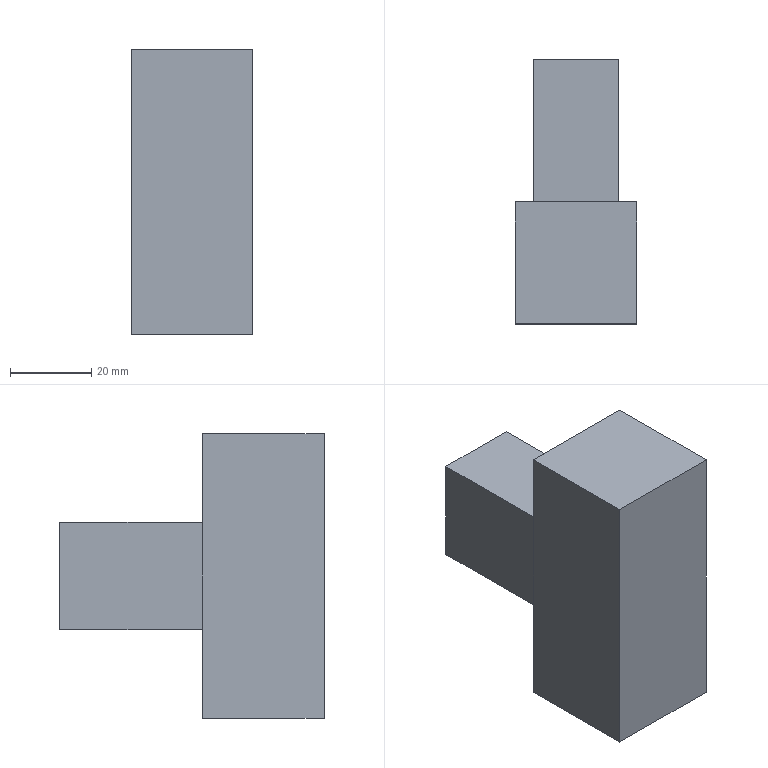Component | SolidWorks | HH54PIntermediateRelay-4 | 1 solid | 11 faces | box 30 x 65 x 70 mm | volume 82477 mm3 | plane 11
build123d program:
from build123d import *

# Parameters (mm, degrees)
SKETCH1_W           = 30
SKETCH1_H           = 70
BOSS_EXTRUDE1_DEPTH = 30
SKETCH2_W           = 21
SKETCH2_H           = 26.5
BOSS_EXTRUDE2_DEPTH = 35


with BuildPart() as part:
    # Sketch1 → Boss-Extrude1 (new body)
    with BuildSketch(Plane.XY):
        with Locations((-5.463, -8.36)):
            Rectangle(SKETCH1_W, SKETCH1_H)
    extrude(amount=BOSS_EXTRUDE1_DEPTH)

    # Sketch2 → Boss-Extrude2 (add)
    with BuildSketch(Plane.XY.offset(30)):
        with Locations((-5.463, -8.36)):
            Rectangle(SKETCH2_W, SKETCH2_H)
    extrude(amount=BOSS_EXTRUDE2_DEPTH)


solid = part.part

# Placed as in the assembly
solid = solid.moved(Location((276.983, -49.298, 757.449), (-90, 0, 0)))
STEP:
#1=COLOUR_RGB('',0.7922,0.8196,0.9333);
#2=FILL_AREA_STYLE_COLOUR('',#1);
#3=FILL_AREA_STYLE('',(#2));
#4=SURFACE_STYLE_FILL_AREA(#3);
#5=SURFACE_SIDE_STYLE('',(#4));
#6=SURFACE_STYLE_USAGE(.BOTH.,#5);
#7=PRESENTATION_STYLE_ASSIGNMENT((#6));
#8=CARTESIAN_POINT('',(10.099,-0.7598,28.772));
#9=VERTEX_POINT('',#8);
#10=CARTESIAN_POINT('',(10.099,-0.7598,31.528));
#11=VERTEX_POINT('',#10);
#12=CARTESIAN_POINT('',(10.099,-0.7598,28.772));
#13=DIRECTION('',(0.,0.,1.));
#14=VECTOR('',#13,39.37);
#15=LINE('',#12,#14);
#16=EDGE_CURVE('',#9,#11,#15,.T.);
#17=ORIENTED_EDGE('',*,*,#16,.T.);
#18=CARTESIAN_POINT('',(11.28,-0.7598,31.528));
#19=VERTEX_POINT('',#18);
#20=CARTESIAN_POINT('',(10.099,-0.7598,31.528));
#21=DIRECTION('',(1.,0.,0.));
#22=VECTOR('',#21,39.37);
#23=LINE('',#20,#22);
#24=EDGE_CURVE('',#11,#19,#23,.T.);
#25=ORIENTED_EDGE('',*,*,#24,.T.);
#26=CARTESIAN_POINT('',(11.28,-0.7598,28.772));
#27=VERTEX_POINT('',#26);
#28=CARTESIAN_POINT('',(11.28,-0.7598,28.772));
#29=DIRECTION('',(-0.,-0.,-1.));
#30=VECTOR('',#29,39.37);
#31=LINE('',#28,#30);
#32=EDGE_CURVE('',#19,#27,#31,.T.);
#33=ORIENTED_EDGE('',*,*,#32,.T.);
#34=CARTESIAN_POINT('',(10.099,-0.7598,28.772));
#35=DIRECTION('',(-1.,0.,0.));
#36=VECTOR('',#35,39.37);
#37=LINE('',#34,#36);
#38=EDGE_CURVE('',#27,#9,#37,.T.);
#39=ORIENTED_EDGE('',*,*,#38,.T.);
#40=EDGE_LOOP('',(#17,#25,#33,#39));
#41=FACE_OUTER_BOUND('',#40,.T.);
#42=CARTESIAN_POINT('',(10.276,-0.7598,30.672));
#43=VERTEX_POINT('',#42);
#44=CARTESIAN_POINT('',(11.103,-0.7598,30.672));
#45=VERTEX_POINT('',#44);
#46=CARTESIAN_POINT('',(10.276,-0.7598,30.672));
#47=DIRECTION('',(1.,0.,0.));
#48=VECTOR('',#47,39.37);
#49=LINE('',#46,#48);
#50=EDGE_CURVE('',#43,#45,#49,.T.);
#51=ORIENTED_EDGE('',*,*,#50,.F.);
#52=CARTESIAN_POINT('',(10.276,-0.7598,29.628));
#53=VERTEX_POINT('',#52);
#54=CARTESIAN_POINT('',(10.276,-0.7598,29.628));
#55=DIRECTION('',(0.,0.,1.));
#56=VECTOR('',#55,39.37);
#57=LINE('',#54,#56);
#58=EDGE_CURVE('',#53,#43,#57,.T.);
#59=ORIENTED_EDGE('',*,*,#58,.F.);
#60=CARTESIAN_POINT('',(11.103,-0.7598,29.628));
#61=VERTEX_POINT('',#60);
#62=CARTESIAN_POINT('',(10.276,-0.7598,29.628));
#63=DIRECTION('',(-1.,0.,0.));
#64=VECTOR('',#63,39.37);
#65=LINE('',#62,#64);
#66=EDGE_CURVE('',#61,#53,#65,.T.);
#67=ORIENTED_EDGE('',*,*,#66,.F.);
#68=CARTESIAN_POINT('',(11.103,-0.7598,29.628));
#69=DIRECTION('',(-0.,-0.,-1.));
#70=VECTOR('',#69,39.37);
#71=LINE('',#68,#70);
#72=EDGE_CURVE('',#45,#61,#71,.T.);
#73=ORIENTED_EDGE('',*,*,#72,.F.);
#74=EDGE_LOOP('',(#51,#59,#67,#73));
#75=FACE_BOUND('',#74,.T.);
#76=CARTESIAN_POINT('',(10.905,-0.7598,29.821));
#77=DIRECTION('',(0.,1.,-0.));
#78=DIRECTION('',(1.,0.,0.));
#79=AXIS2_PLACEMENT_3D('',#76,#77,#78);
#80=PLANE('',#79);
#81=ADVANCED_FACE('',(#41,#75),#80,.T.);
#82=CARTESIAN_POINT('',(10.099,-1.941,28.772));
#83=VERTEX_POINT('',#82);
#84=CARTESIAN_POINT('',(10.099,-1.941,31.528));
#85=VERTEX_POINT('',#84);
#86=CARTESIAN_POINT('',(10.099,-1.941,28.772));
#87=DIRECTION('',(0.,0.,1.));
#88=VECTOR('',#87,39.37);
#89=LINE('',#86,#88);
#90=EDGE_CURVE('',#83,#85,#89,.T.);
#91=ORIENTED_EDGE('',*,*,#90,.T.);
#92=CARTESIAN_POINT('',(10.099,-0.7598,31.528));
#93=DIRECTION('',(0.,-1.,0.));
#94=VECTOR('',#93,39.37);
#95=LINE('',#92,#94);
#96=EDGE_CURVE('',#11,#85,#95,.T.);
#97=ORIENTED_EDGE('',*,*,#96,.F.);
#98=ORIENTED_EDGE('',*,*,#16,.F.);
#99=CARTESIAN_POINT('',(10.099,-0.7598,28.772));
#100=DIRECTION('',(0.,-1.,0.));
#101=VECTOR('',#100,39.37);
#102=LINE('',#99,#101);
#103=EDGE_CURVE('',#9,#83,#102,.T.);
#104=ORIENTED_EDGE('',*,*,#103,.T.);
#105=EDGE_LOOP('',(#91,#97,#98,#104));
#106=FACE_OUTER_BOUND('',#105,.T.);
#107=CARTESIAN_POINT('',(10.099,-0.7598,28.772));
#108=DIRECTION('',(1.,0.,0.));
#109=DIRECTION('',(0.,-1.,0.));
#110=AXIS2_PLACEMENT_3D('',#107,#108,#109);
#111=PLANE('',#110);
#112=ADVANCED_FACE('',(#106),#111,.F.);
#113=CARTESIAN_POINT('',(11.28,-1.941,31.528));
#114=VERTEX_POINT('',#113);
#115=CARTESIAN_POINT('',(10.099,-1.941,31.528));
#116=DIRECTION('',(1.,0.,0.));
#117=VECTOR('',#116,39.37);
#118=LINE('',#115,#117);
#119=EDGE_CURVE('',#85,#114,#118,.T.);
#120=ORIENTED_EDGE('',*,*,#119,.T.);
#121=CARTESIAN_POINT('',(11.28,-0.7598,31.528));
#122=DIRECTION('',(0.,-1.,0.));
#123=VECTOR('',#122,39.37);
#124=LINE('',#121,#123);
#125=EDGE_CURVE('',#19,#114,#124,.T.);
#126=ORIENTED_EDGE('',*,*,#125,.F.);
#127=ORIENTED_EDGE('',*,*,#24,.F.);
#128=ORIENTED_EDGE('',*,*,#96,.T.);
#129=EDGE_LOOP('',(#120,#126,#127,#128));
#130=FACE_OUTER_BOUND('',#129,.T.);
#131=CARTESIAN_POINT('',(10.099,-0.7598,31.528));
#132=DIRECTION('',(0.,-0.,-1.));
#133=DIRECTION('',(0.,1.,-0.));
#134=AXIS2_PLACEMENT_3D('',#131,#132,#133);
#135=PLANE('',#134);
#136=ADVANCED_FACE('',(#130),#135,.F.);
#137=CARTESIAN_POINT('',(11.28,-1.941,28.772));
#138=VERTEX_POINT('',#137);
#139=CARTESIAN_POINT('',(11.28,-1.941,28.772));
#140=DIRECTION('',(-0.,-0.,-1.));
#141=VECTOR('',#140,39.37);
#142=LINE('',#139,#141);
#143=EDGE_CURVE('',#114,#138,#142,.T.);
#144=ORIENTED_EDGE('',*,*,#143,.T.);
#145=CARTESIAN_POINT('',(11.28,-0.7598,28.772));
#146=DIRECTION('',(0.,-1.,0.));
#147=VECTOR('',#146,39.37);
#148=LINE('',#145,#147);
#149=EDGE_CURVE('',#27,#138,#148,.T.);
#150=ORIENTED_EDGE('',*,*,#149,.F.);
#151=ORIENTED_EDGE('',*,*,#32,.F.);
#152=ORIENTED_EDGE('',*,*,#125,.T.);
#153=EDGE_LOOP('',(#144,#150,#151,#152));
#154=FACE_OUTER_BOUND('',#153,.T.);
#155=CARTESIAN_POINT('',(11.28,-0.7598,28.772));
#156=DIRECTION('',(-1.,0.,0.));
#157=DIRECTION('',(0.,0.,1.));
#158=AXIS2_PLACEMENT_3D('',#155,#156,#157);
#159=PLANE('',#158);
#160=ADVANCED_FACE('',(#154),#159,.F.);
#161=CARTESIAN_POINT('',(10.099,-1.941,28.772));
#162=DIRECTION('',(-1.,0.,0.));
#163=VECTOR('',#162,39.37);
#164=LINE('',#161,#163);
#165=EDGE_CURVE('',#138,#83,#164,.T.);
#166=ORIENTED_EDGE('',*,*,#165,.T.);
#167=ORIENTED_EDGE('',*,*,#103,.F.);
#168=ORIENTED_EDGE('',*,*,#38,.F.);
#169=ORIENTED_EDGE('',*,*,#149,.T.);
#170=EDGE_LOOP('',(#166,#167,#168,#169));
#171=FACE_OUTER_BOUND('',#170,.T.);
#172=CARTESIAN_POINT('',(10.099,-0.7598,28.772));
#173=DIRECTION('',(0.,0.,1.));
#174=DIRECTION('',(0.,-1.,0.));
#175=AXIS2_PLACEMENT_3D('',#172,#173,#174);
#176=PLANE('',#175);
#177=ADVANCED_FACE('',(#171),#176,.F.);
#178=ORIENTED_EDGE('',*,*,#90,.F.);
#179=ORIENTED_EDGE('',*,*,#165,.F.);
#180=ORIENTED_EDGE('',*,*,#143,.F.);
#181=ORIENTED_EDGE('',*,*,#119,.F.);
#182=EDGE_LOOP('',(#178,#179,#180,#181));
#183=FACE_OUTER_BOUND('',#182,.T.);
#184=CARTESIAN_POINT('',(10.905,-1.941,29.821));
#185=DIRECTION('',(0.,1.,-0.));
#186=DIRECTION('',(1.,0.,0.));
#187=AXIS2_PLACEMENT_3D('',#184,#185,#186);
#188=PLANE('',#187);
#189=ADVANCED_FACE('',(#183),#188,.F.);
#190=ORIENTED_EDGE('',*,*,#58,.T.);
#191=CARTESIAN_POINT('',(10.276,0.6182,30.672));
#192=VERTEX_POINT('',#191);
#193=CARTESIAN_POINT('',(10.276,0.6182,30.672));
#194=DIRECTION('',(0.,-1.,0.));
#195=VECTOR('',#194,39.37);
#196=LINE('',#193,#195);
#197=EDGE_CURVE('',#192,#43,#196,.T.);
#198=ORIENTED_EDGE('',*,*,#197,.F.);
#199=CARTESIAN_POINT('',(10.276,0.6182,29.628));
#200=VERTEX_POINT('',#199);
#201=CARTESIAN_POINT('',(10.276,0.6182,29.628));
#202=DIRECTION('',(0.,0.,1.));
#203=VECTOR('',#202,39.37);
#204=LINE('',#201,#203);
#205=EDGE_CURVE('',#200,#192,#204,.T.);
#206=ORIENTED_EDGE('',*,*,#205,.F.);
#207=CARTESIAN_POINT('',(10.276,0.6182,29.628));
#208=DIRECTION('',(0.,-1.,0.));
#209=VECTOR('',#208,39.37);
#210=LINE('',#207,#209);
#211=EDGE_CURVE('',#200,#53,#210,.T.);
#212=ORIENTED_EDGE('',*,*,#211,.T.);
#213=EDGE_LOOP('',(#190,#198,#206,#212));
#214=FACE_OUTER_BOUND('',#213,.T.);
#215=CARTESIAN_POINT('',(10.276,0.6182,29.628));
#216=DIRECTION('',(1.,-0.,-0.));
#217=DIRECTION('',(-0.,-0.,-1.));
#218=AXIS2_PLACEMENT_3D('',#215,#216,#217);
#219=PLANE('',#218);
#220=ADVANCED_FACE('',(#214),#219,.F.);
#221=ORIENTED_EDGE('',*,*,#50,.T.);
#222=CARTESIAN_POINT('',(11.103,0.6182,30.672));
#223=VERTEX_POINT('',#222);
#224=CARTESIAN_POINT('',(11.103,0.6182,30.672));
#225=DIRECTION('',(0.,-1.,0.));
#226=VECTOR('',#225,39.37);
#227=LINE('',#224,#226);
#228=EDGE_CURVE('',#223,#45,#227,.T.);
#229=ORIENTED_EDGE('',*,*,#228,.F.);
#230=CARTESIAN_POINT('',(10.276,0.6182,30.672));
#231=DIRECTION('',(1.,0.,0.));
#232=VECTOR('',#231,39.37);
#233=LINE('',#230,#232);
#234=EDGE_CURVE('',#192,#223,#233,.T.);
#235=ORIENTED_EDGE('',*,*,#234,.F.);
#236=ORIENTED_EDGE('',*,*,#197,.T.);
#237=EDGE_LOOP('',(#221,#229,#235,#236));
#238=FACE_OUTER_BOUND('',#237,.T.);
#239=CARTESIAN_POINT('',(10.276,0.6182,30.672));
#240=DIRECTION('',(0.,-0.,-1.));
#241=DIRECTION('',(-1.,-0.,-0.));
#242=AXIS2_PLACEMENT_3D('',#239,#240,#241);
#243=PLANE('',#242);
#244=ADVANCED_FACE('',(#238),#243,.F.);
#245=ORIENTED_EDGE('',*,*,#72,.T.);
#246=CARTESIAN_POINT('',(11.103,0.6182,29.628));
#247=VERTEX_POINT('',#246);
#248=CARTESIAN_POINT('',(11.103,0.6182,29.628));
#249=DIRECTION('',(0.,-1.,0.));
#250=VECTOR('',#249,39.37);
#251=LINE('',#248,#250);
#252=EDGE_CURVE('',#247,#61,#251,.T.);
#253=ORIENTED_EDGE('',*,*,#252,.F.);
#254=CARTESIAN_POINT('',(11.103,0.6182,29.628));
#255=DIRECTION('',(-0.,-0.,-1.));
#256=VECTOR('',#255,39.37);
#257=LINE('',#254,#256);
#258=EDGE_CURVE('',#223,#247,#257,.T.);
#259=ORIENTED_EDGE('',*,*,#258,.F.);
#260=ORIENTED_EDGE('',*,*,#228,.T.);
#261=EDGE_LOOP('',(#245,#253,#259,#260));
#262=FACE_OUTER_BOUND('',#261,.T.);
#263=CARTESIAN_POINT('',(11.103,0.6182,29.628));
#264=DIRECTION('',(-1.,0.,0.));
#265=DIRECTION('',(0.,0.,1.));
#266=AXIS2_PLACEMENT_3D('',#263,#264,#265);
#267=PLANE('',#266);
#268=ADVANCED_FACE('',(#262),#267,.F.);
#269=ORIENTED_EDGE('',*,*,#66,.T.);
#270=ORIENTED_EDGE('',*,*,#211,.F.);
#271=CARTESIAN_POINT('',(10.276,0.6182,29.628));
#272=DIRECTION('',(-1.,0.,0.));
#273=VECTOR('',#272,39.37);
#274=LINE('',#271,#273);
#275=EDGE_CURVE('',#247,#200,#274,.T.);
#276=ORIENTED_EDGE('',*,*,#275,.F.);
#277=ORIENTED_EDGE('',*,*,#252,.T.);
#278=EDGE_LOOP('',(#269,#270,#276,#277));
#279=FACE_OUTER_BOUND('',#278,.T.);
#280=CARTESIAN_POINT('',(10.276,0.6182,29.628));
#281=DIRECTION('',(0.,0.,1.));
#282=DIRECTION('',(0.,-1.,0.));
#283=AXIS2_PLACEMENT_3D('',#280,#281,#282);
#284=PLANE('',#283);
#285=ADVANCED_FACE('',(#279),#284,.F.);
#286=ORIENTED_EDGE('',*,*,#205,.T.);
#287=ORIENTED_EDGE('',*,*,#234,.T.);
#288=ORIENTED_EDGE('',*,*,#258,.T.);
#289=ORIENTED_EDGE('',*,*,#275,.T.);
#290=EDGE_LOOP('',(#286,#287,#288,#289));
#291=FACE_OUTER_BOUND('',#290,.T.);
#292=CARTESIAN_POINT('',(10.905,0.6182,29.821));
#293=DIRECTION('',(0.,1.,-0.));
#294=DIRECTION('',(1.,0.,0.));
#295=AXIS2_PLACEMENT_3D('',#292,#293,#294);
#296=PLANE('',#295);
#297=ADVANCED_FACE('',(#291),#296,.T.);
#298=CLOSED_SHELL('',(#81,#112,#136,#160,#177,#189,#220,#244,#268,#285,#297));
#299=MANIFOLD_SOLID_BREP('',#298);
#300=STYLED_ITEM('',(#7),#299);
#301=PRESENTATION_LAYER_ASSIGNMENT('','',(#300));
#302=(LENGTH_UNIT()NAMED_UNIT(*)SI_UNIT($,.METRE.));
#303=LENGTH_MEASURE_WITH_UNIT(LENGTH_MEASURE(0.0254),#302);
#304=DIMENSIONAL_EXPONENTS(1.,0.,0.,0.,0.,0.,0.);
#305=(CONVERSION_BASED_UNIT('',#303)LENGTH_UNIT()NAMED_UNIT(#304));
#306=UNCERTAINTY_MEASURE_WITH_UNIT(LENGTH_MEASURE(0.00001),#305,'','');
#307=(NAMED_UNIT(*)PLANE_ANGLE_UNIT()SI_UNIT($,.RADIAN.));
#308=(NAMED_UNIT(*)SI_UNIT($,.STERADIAN.)SOLID_ANGLE_UNIT());
#309=(GEOMETRIC_REPRESENTATION_CONTEXT(3)GLOBAL_UNCERTAINTY_ASSIGNED_CONTEXT((#306))GLOBAL_UNIT_ASSIGNED_CONTEXT((#305,#307,#308))REPRESENTATION_CONTEXT('',''));
#310=MECHANICAL_DESIGN_GEOMETRIC_PRESENTATION_REPRESENTATION('',(#300),#309);
#311=CARTESIAN_POINT('',(0.,0.,0.));
#312=DIRECTION('',(0.,0.,1.));
#313=DIRECTION('',(1.,0.,0.));
#314=AXIS2_PLACEMENT_3D('',#311,#312,#313);
#315=(LENGTH_UNIT()NAMED_UNIT(*)SI_UNIT($,.METRE.));
#316=LENGTH_MEASURE_WITH_UNIT(LENGTH_MEASURE(0.0254),#315);
#317=DIMENSIONAL_EXPONENTS(1.,0.,0.,0.,0.,0.,0.);
#318=(CONVERSION_BASED_UNIT('',#316)LENGTH_UNIT()NAMED_UNIT(#317));
#319=UNCERTAINTY_MEASURE_WITH_UNIT(LENGTH_MEASURE(0.00001),#318,'','');
#320=(NAMED_UNIT(*)PLANE_ANGLE_UNIT()SI_UNIT($,.RADIAN.));
#321=(NAMED_UNIT(*)SI_UNIT($,.STERADIAN.)SOLID_ANGLE_UNIT());
#322=(GEOMETRIC_REPRESENTATION_CONTEXT(3)GLOBAL_UNCERTAINTY_ASSIGNED_CONTEXT((#319))GLOBAL_UNIT_ASSIGNED_CONTEXT((#318,#320,#321))REPRESENTATION_CONTEXT('',''));
#323=ADVANCED_BREP_SHAPE_REPRESENTATION('',(#299,#314),#322);